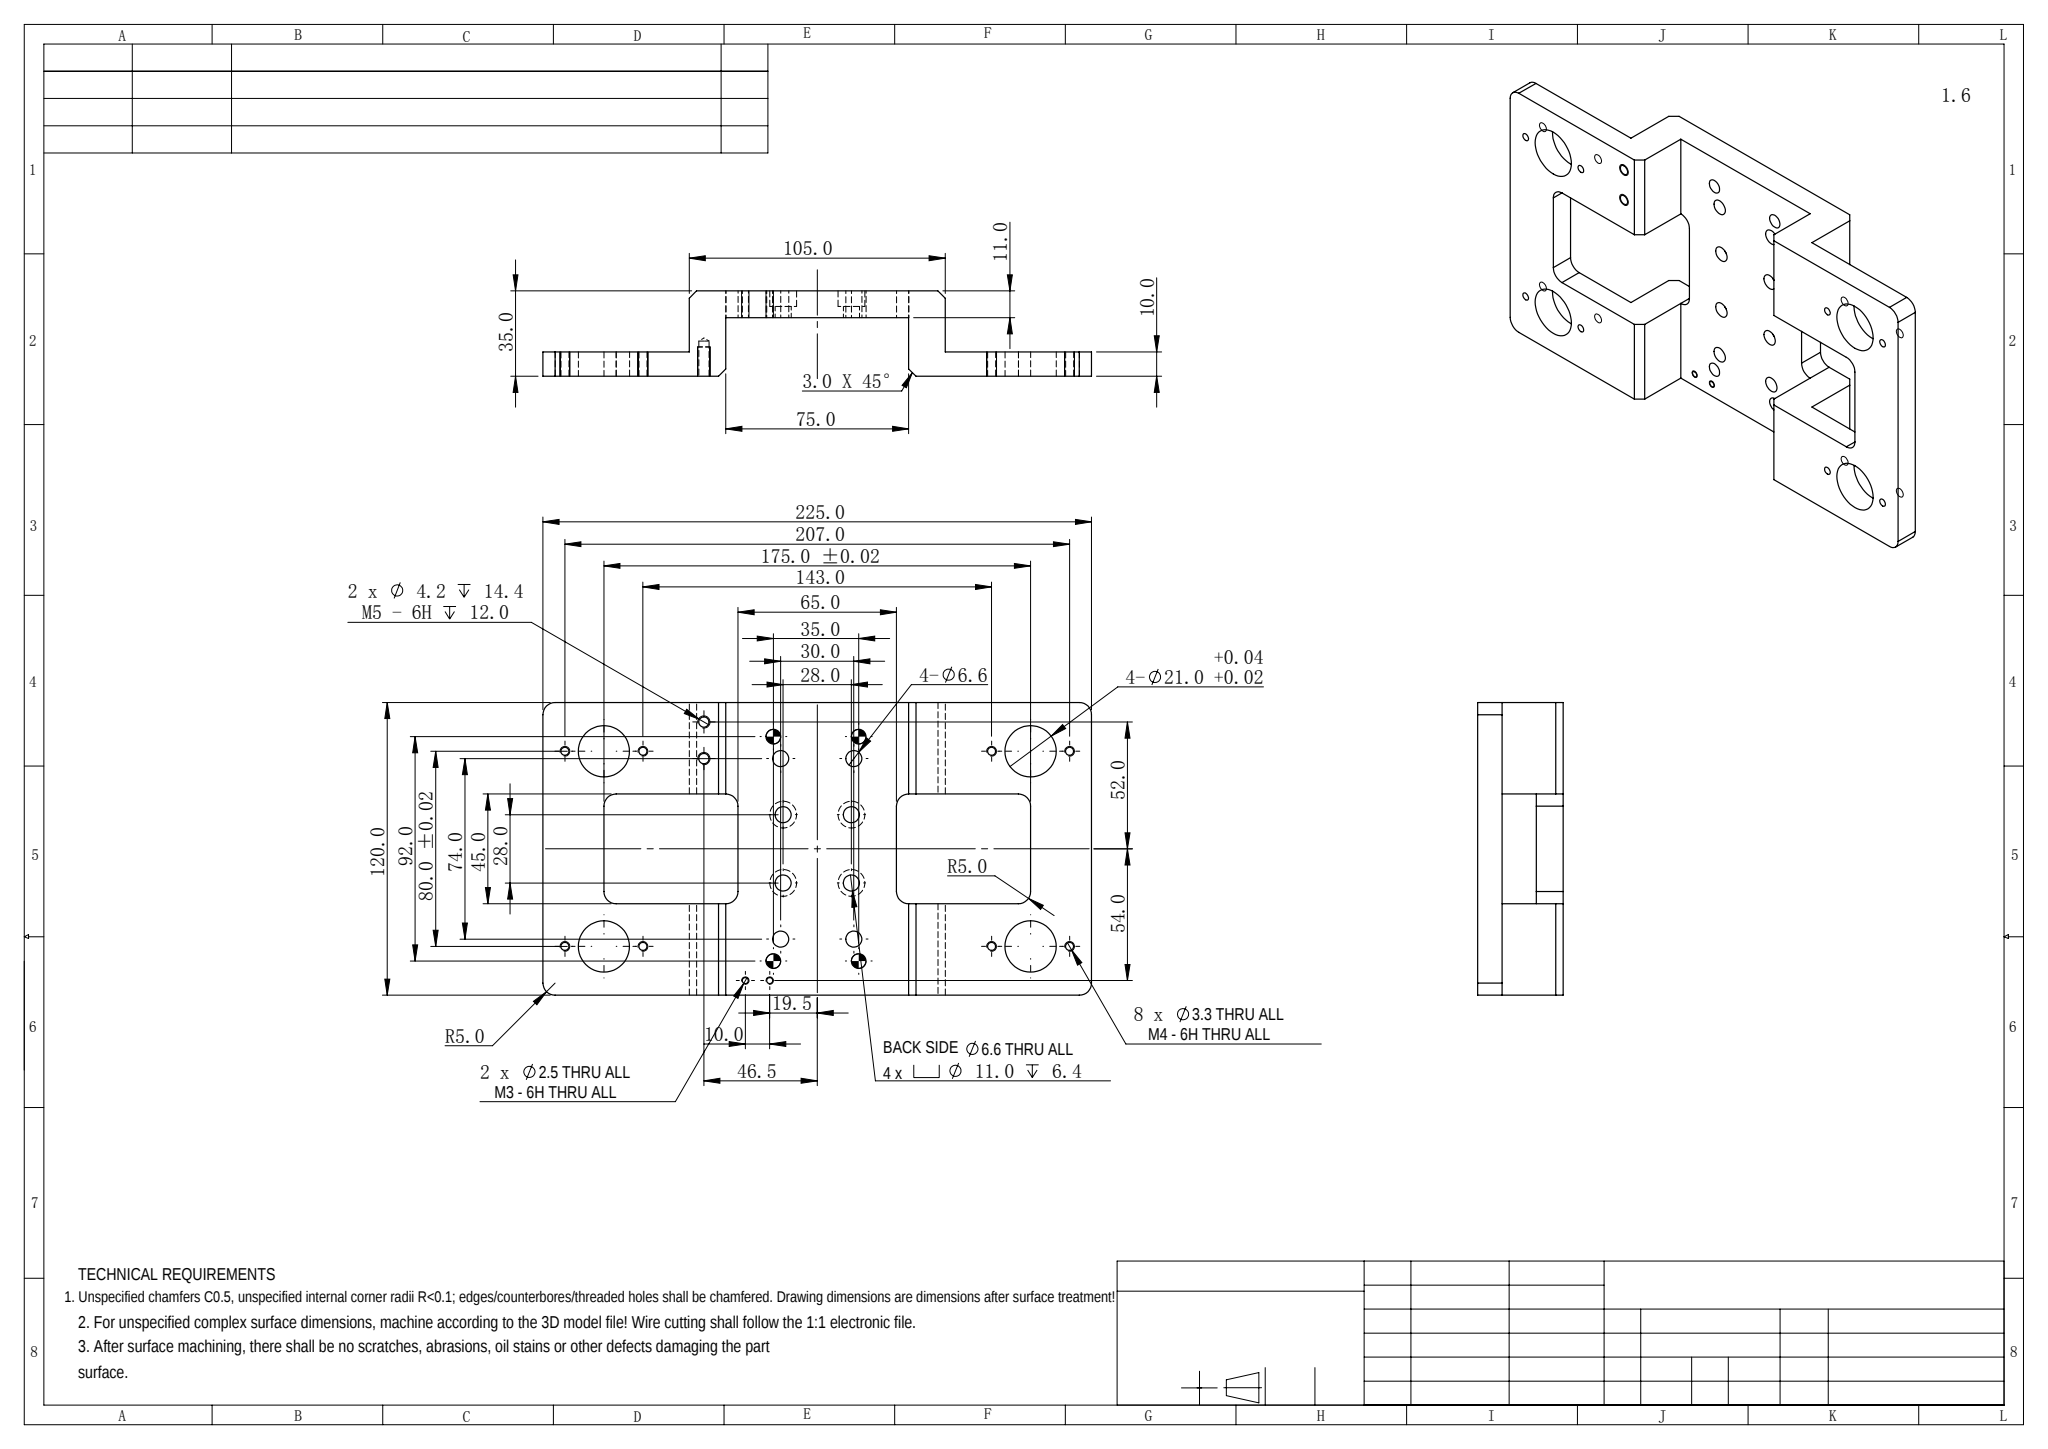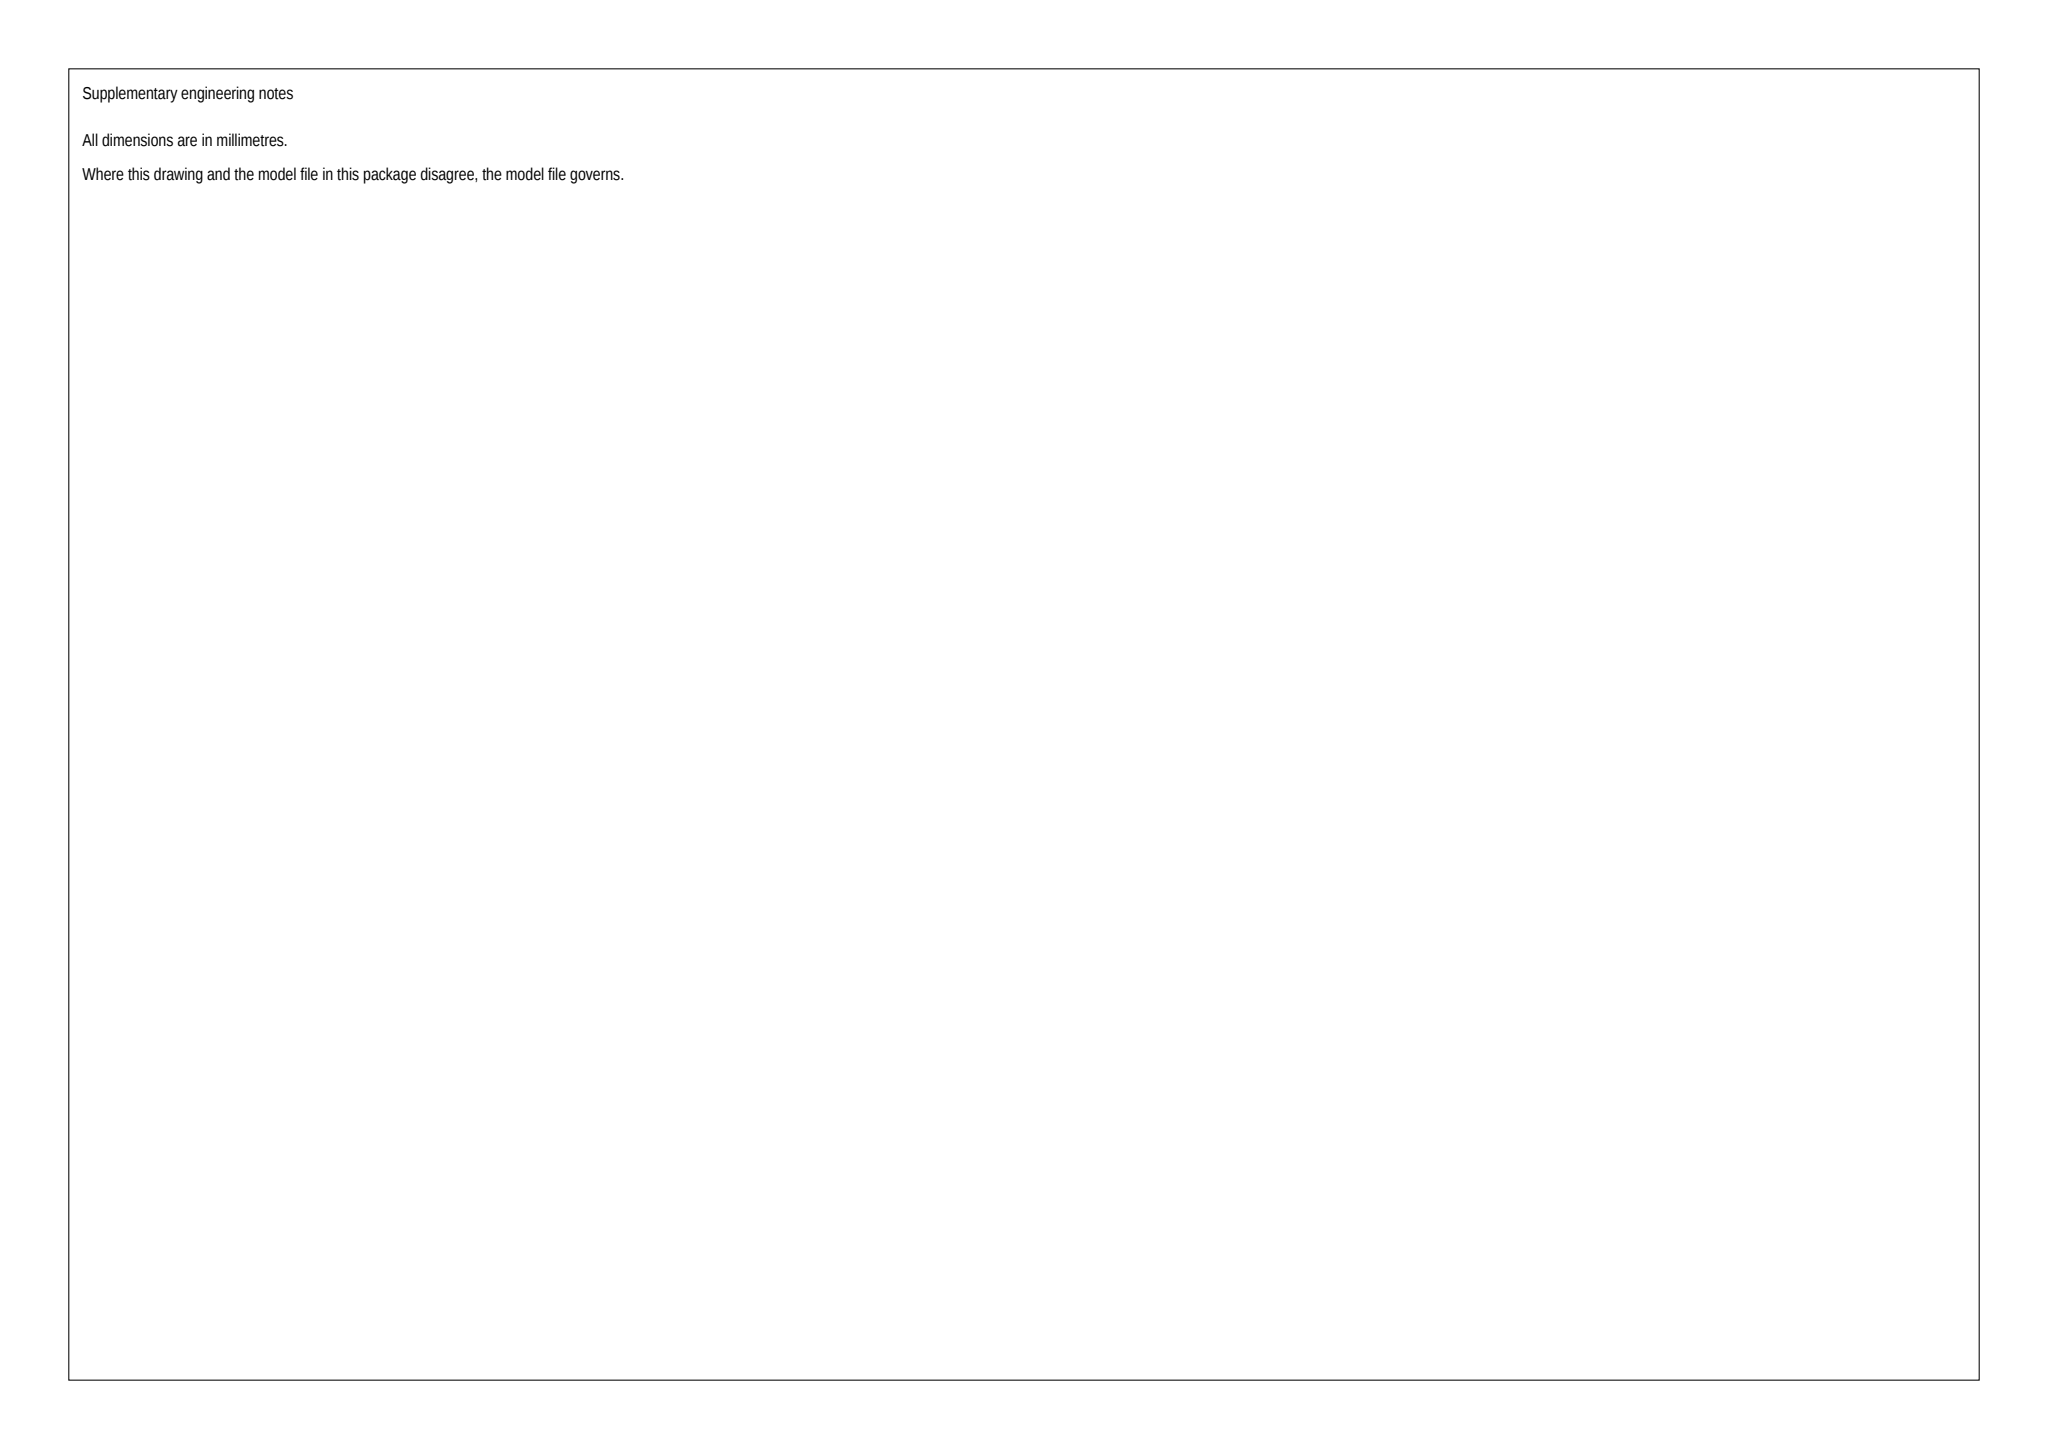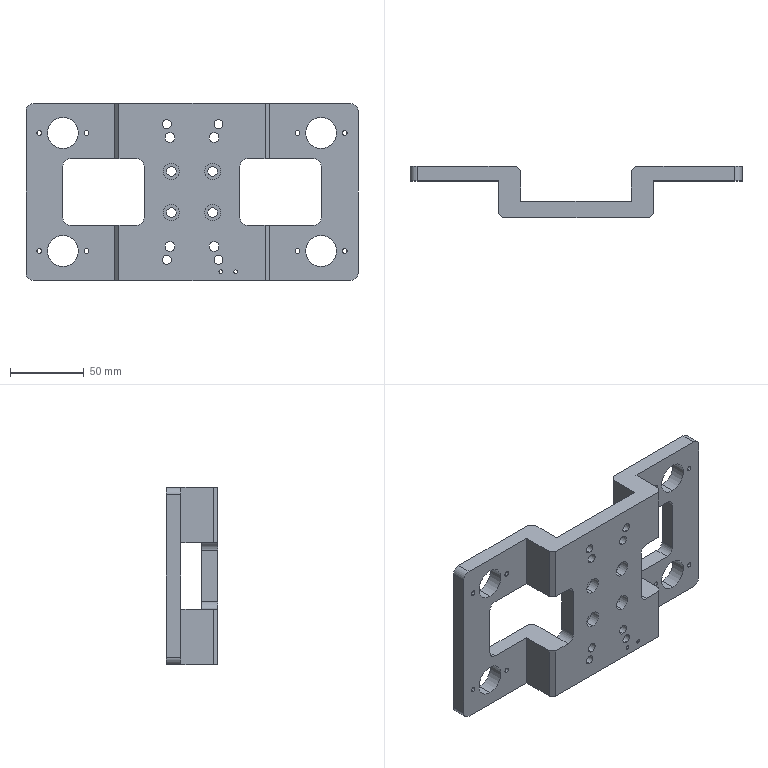Part | SolidWorks | mm | 1 solid | 118 faces | box 225 x 35 x 120 mm | volume 263317 mm3 | cylinder 76 | plane 38 | cone 4 | commonest cylinder face diameters 3.3 x16 6.6 x16 10 x12 11 x8 6 x8 21 x8 4.2 x4 2.5 x4
Drawing notes:
OVERALL 225 X 120 X 35 | from the solid: bbox_xyz 225/120/35
STEPPED PROFILE: STEPS Z=37.5 & 82.5 FROM BTM; FACES Y=11 & 25 FROM FRONT | from the solid: z planes 0/37.5/82.5/120; y planes 0/11/25/35
2X WINDOW 55 X 45 R5 CNRS THRU; X=25 & 145, Z=37.5 FROM LH/BTM | from the solid: x planes 25/80 & 145/200, z 37.5/82.5; R5 cnr cyls Ø10 at (30,42.5)(75,77.5)(150,-)(195,-) thru
4X Ø21 +0.04/+0.02 THRU AT X=25 & 200, Z=20 & 100 FROM LH/BTM | from the solid: cyl dia21 axis y at [25,20][25,100][200,20][200,100], len 10
4X Ø6 THRU AT X=95.5 & 130.5, Z=14 & 106 FROM LH/BTM | from the solid: cyl dia6.0 axis y len 11 at [95.5,14][95.5,106][130.5,14][130.5,106]
4X Ø6.6 THRU AT X=97.5 & 127.5, Z=23 & 97 FROM LH/BTM | from the solid: cyl dia6.6 axis y len 11 at [97.5,23][97.5,97][127.5,23][127.5,97]
4X Ø6.6 THRU, CBORE Ø11 DP6.4 BACK SIDE; X=98.5 & 126.5, Z=46 & 74 | from the solid: Ø11 len 6.4 + Ø6.6 len 4.6 coaxial at [98.5,46][98.5,74][126.5,46][126.5,74]; y plane 6.4 x4
8X Ø3.3 M4-6H THRU AT X=9,41,184,216; Z=20 & 100 FROM LH/BTM | from the solid: cyl dia3.3 axis y len 10 at x=9,41,184,216 with z=20 and z=100
2X Ø4.2 DP14.4, M5-6H DP12 AT X=159, Z=97 & 112 FROM LH/BTM | from the solid: dia4.2 len14.4 at [159,97][159,112]; cone 118 ref dia 4.2
2X Ø2.5 M3-6H THRU AT X=132 & 142, Z=6 FROM LH/BTM | from the solid: cyl dia2.5 axis y len 11 at [132,6][142,6]
4X Ø6.6 THRU, CBORE Ø11 DP6.4 FROM BACK SIDE, AT X=98.5 & 126.5, Z=46 & 74 FROM LH/BTM | from the solid: cylinders dia 6.6 len 4.6 at (98.5/126.5, z=46/74) with dia 11 len 6.4 coaxial; y-plane offset 6.4
8X Ø3.3 M4-6H THRU AT X=9, 41, 184 & 216, Z=20 & 100 FROM LH/BTM | from the solid: cylinders dia 3.3 axis y len 10 at x=9,41,184,216 and z=20,100
build123d program:
from build123d import *

# Parameters (mm, degrees)
SKETCH1_W                                       = 225
SKETCH1_H                                       = 120
BOSS_EXTRUDE1_DEPTH                             = 35
FILLET1_R                                       = 5
SKETCH2_R                                       = 10.5
CUT_EXTRUDE1_DEPTH                              = 62
SKETCH3_R                                       = 3
CUT_EXTRUDE2_DEPTH                              = 65
SKETCH4_W                                       = 55
SKETCH4_H                                       = 45
CUT_EXTRUDE3_DEPTH                              = 145
FILLET2_R                                       = 5
M6_HEX_SOCKET_HEAD_CAP_SCREW_CBORE2_D           = 6.6
M6_HEX_SOCKET_HEAD_CAP_SCREW_CBORE2_CBORE_D     = 11
M6_HEX_SOCKET_HEAD_CAP_SCREW_CBORE2_CBORE_DEPTH = 6.4
M6_HEX_SOCKET_HEAD_CAP_SCREW_CBORE1_D           = 6.6
M6_HEX_SOCKET_HEAD_CAP_SCREW_CBORE1_CBORE_D     = 11
M6_HEX_SOCKET_HEAD_CAP_SCREW_CBORE1_CBORE_DEPTH = 6.4
M4_TAPPED_HOLE1_D                               = 3.3
SKETCH17_W                                      = 75
SKETCH17_H                                      = 48
SKETCH17_W_2                                    = 120
SKETCH17_H_2                                    = 50
CUT_EXTRUDE4_DEPTH                              = 169.17
CHAMFER1_SIZE                                   = 3
M3_TAPPED_HOLE1_D                               = 2.5
M5_TAPPED_HOLE3_D                               = 4.2
M5_TAPPED_HOLE3_DEPTH                           = 14.4
M5_TAPPED_HOLE3_TIP                             = 1.262


with BuildPart() as part:
    # Sketch1 → Boss-Extrude1 (new body)
    with BuildSketch(Plane(origin=(0, 0, 0), x_dir=(1, 0, 0), z_dir=(0, 1, 0))):
        Rectangle(SKETCH1_W, SKETCH1_H)
    extrude(amount=BOSS_EXTRUDE1_DEPTH)

    # Fillet1
    fillet1_edges = [part.edges().sort_by_distance(p)[0] for p in [
        (112.5, 17.5, 60),
        (-112.5, 17.5, 60),
        (-112.5, 17.5, -60),
        (112.5, 17.5, -60),
    ]]
    fillet(fillet1_edges, radius=FILLET1_R)

    # Sketch2 → Cut-Extrude1 (cut)
    with BuildSketch(Plane(origin=(0, 35, 0), x_dir=(1, 0, 0), z_dir=(0, 1, 0))):
        with Locations(Location((-87.5, 40, 0), (0, 0, 270))):
            Circle(SKETCH2_R)
        with Locations(Location((87.5, 40, 0), (0, 0, 270))):
            Circle(SKETCH2_R)
        with Locations(Location((87.5, -40, 0), (0, 0, 90))):
            Circle(SKETCH2_R)
        with Locations(Location((-87.5, -40, 0), (0, 0, 90))):
            Circle(SKETCH2_R)
    extrude(amount=-CUT_EXTRUDE1_DEPTH, mode=Mode.SUBTRACT)

    # Sketch3 → Cut-Extrude2 (cut)
    with BuildSketch(Plane(origin=(0, 35, 0), x_dir=(1, 0, 0), z_dir=(0, 1, 0))):
        with Locations(Location((18, -46, 0), (0, 0, 270))):
            Circle(SKETCH3_R)
        with Locations(Location((-17, -46, 0), (0, 0, 270))):
            Circle(SKETCH3_R)
        with Locations(Location((-17, 46, 0), (0, 0, 90))):
            Circle(SKETCH3_R)
        with Locations(Location((18, 46, 0), (0, 0, 90))):
            Circle(SKETCH3_R)
    extrude(amount=-CUT_EXTRUDE2_DEPTH, mode=Mode.SUBTRACT)

    # Sketch4 → Cut-Extrude3 (cut)
    with BuildSketch(Plane(origin=(0, 35, 0), x_dir=(1, 0, 0), z_dir=(0, 1, 0))):
        with Locations((-60, 0)):
            Rectangle(SKETCH4_W, SKETCH4_H)
        with Locations((60, 0)):
            Rectangle(SKETCH4_W, SKETCH4_H)
    extrude(amount=-CUT_EXTRUDE3_DEPTH, mode=Mode.SUBTRACT)

    # Fillet2
    fillet2_edges = [part.edges().sort_by_distance(p)[0] for p in [
        (32.5, 17.5, -22.5),
        (87.5, 17.5, -22.5),
        (87.5, 17.5, 22.5),
        (32.5, 17.5, 22.5),
        (-32.5, 17.5, -22.5),
        (-32.5, 17.5, 22.5),
        (-87.5, 17.5, 22.5),
        (-87.5, 17.5, -22.5),
    ]]
    fillet(fillet2_edges, radius=FILLET2_R)

    # M6 Hex Socket Head Cap Screw CBORE2 (through all)
    with Locations(Plane(origin=(0, 35, 0), x_dir=(1, 0, 0), z_dir=(0, 1, 0))):
        with Locations((-15, 37), (15, 37), (15, -37), (-15, -37)):
            CounterBoreHole(M6_HEX_SOCKET_HEAD_CAP_SCREW_CBORE2_D / 2, M6_HEX_SOCKET_HEAD_CAP_SCREW_CBORE2_CBORE_D / 2, M6_HEX_SOCKET_HEAD_CAP_SCREW_CBORE2_CBORE_DEPTH)

    # M6 Hex Socket Head Cap Screw CBORE1 (through all)
    with Locations(Plane(origin=(0, 0, 0), x_dir=(-1, 0, 0), z_dir=(0, -1, 0))):
        with Locations((14, 14), (14, -14), (-14, -14), (-14, 14)):
            CounterBoreHole(M6_HEX_SOCKET_HEAD_CAP_SCREW_CBORE1_D / 2, M6_HEX_SOCKET_HEAD_CAP_SCREW_CBORE1_CBORE_D / 2, M6_HEX_SOCKET_HEAD_CAP_SCREW_CBORE1_CBORE_DEPTH)

    # M4 Tapped Hole1 (through all)
    with Locations(Plane(origin=(0, 0, 0), x_dir=(-1, 0, 0), z_dir=(0, -1, 0))):
        with Locations((-71.5, 40), (-103.5, 40), (-71.5, -40), (-103.5, -40), (71.5, -40), (103.5, -40), (103.5, 40), (71.5, 40)):
            Hole(M4_TAPPED_HOLE1_D / 2)

    # Sketch17 → Cut-Extrude4 (cut, through all)
    with BuildSketch(Plane.XY.offset(60)):
        with Locations((0, 35)):
            Rectangle(SKETCH17_W, SKETCH17_H)
        with Locations((-112.5, 0)):
            Rectangle(SKETCH17_W_2, SKETCH17_H_2)
        with Locations((112.5, 0)):
            Rectangle(SKETCH17_W_2, SKETCH17_H_2)
    extrude(amount=-CUT_EXTRUDE4_DEPTH, mode=Mode.SUBTRACT)

    # Chamfer1
    chamfer1_edges = [part.edges().sort_by_distance(p)[0] for p in [
        (37.5, 35, -41.25),
        (37.5, 35, 41.25),
        (-37.5, 35, -41.25),
        (-37.5, 35, 41.25),
        (-52.5, 0, 41.25),
        (-52.5, 0, -41.25),
        (52.5, 0, -41.25),
        (52.5, 0, 41.25),
    ]]
    chamfer(chamfer1_edges, length=CHAMFER1_SIZE)

    # M3 Tapped Hole1 (through all)
    with Locations(Plane(origin=(0, 11, 0), x_dir=(1, 0, 0), z_dir=(0, 1, 0))):
        with Locations((29.5, 54), (19.5, 54)):
            Hole(M3_TAPPED_HOLE1_D / 2)

    # M5 Tapped Hole3
    with Locations(Plane(origin=(0, 35, 0), x_dir=(1, 0, 0), z_dir=(0, 1, 0))):
        with Locations((46.5, -37), (46.5, -52)):
            Hole(M5_TAPPED_HOLE3_D / 2, depth=M5_TAPPED_HOLE3_DEPTH)
            with Locations((0, 0, -(M5_TAPPED_HOLE3_DEPTH + M5_TAPPED_HOLE3_TIP / 2))):  # 118° drill point
                Cone(0, M5_TAPPED_HOLE3_D / 2, M5_TAPPED_HOLE3_TIP, mode=Mode.SUBTRACT)


solid = part.part